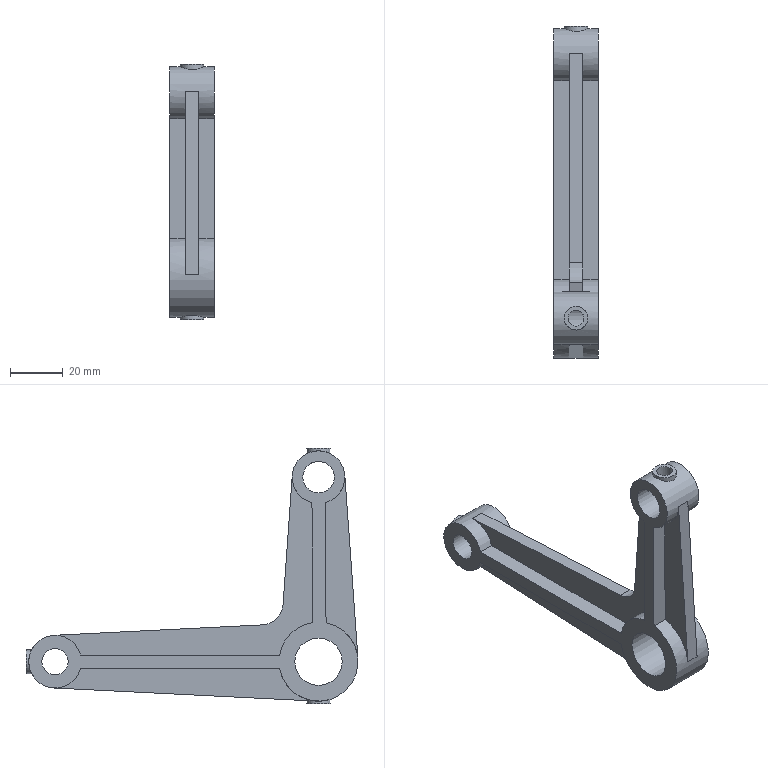Component | NX | PRODUCT | 1 solid | 37 faces | volume 38302 mm3 | plane 23 | cylinder 14 | commonest cylinder face diameters 30 x3 9 x3 20 x2 6 x2 16 x1 18 x1 12 x1 10 x1